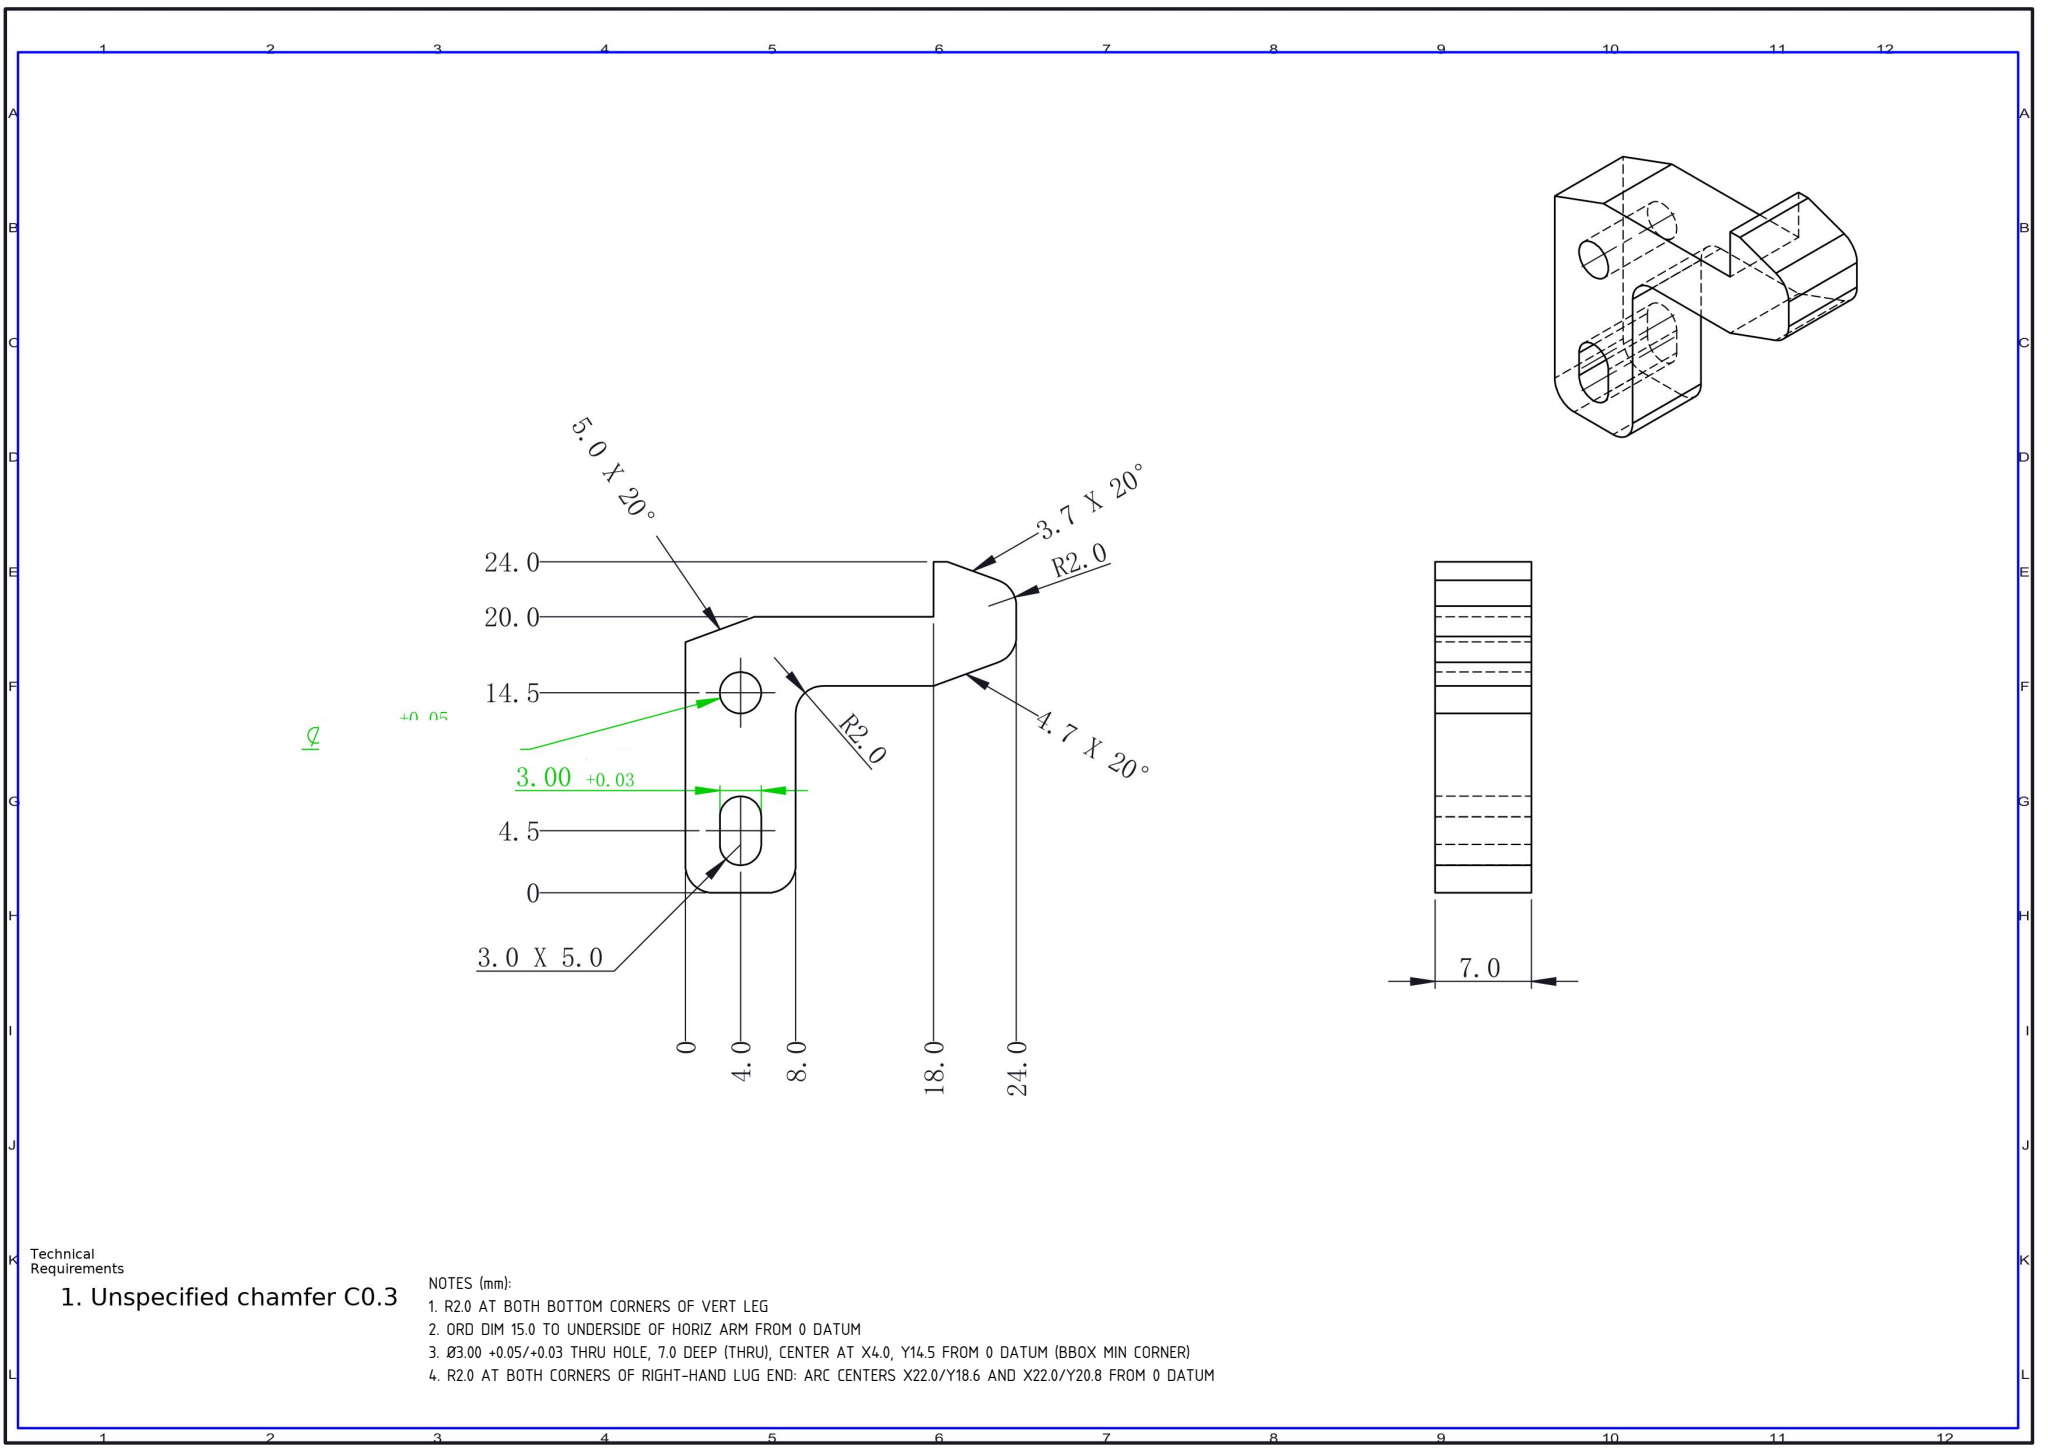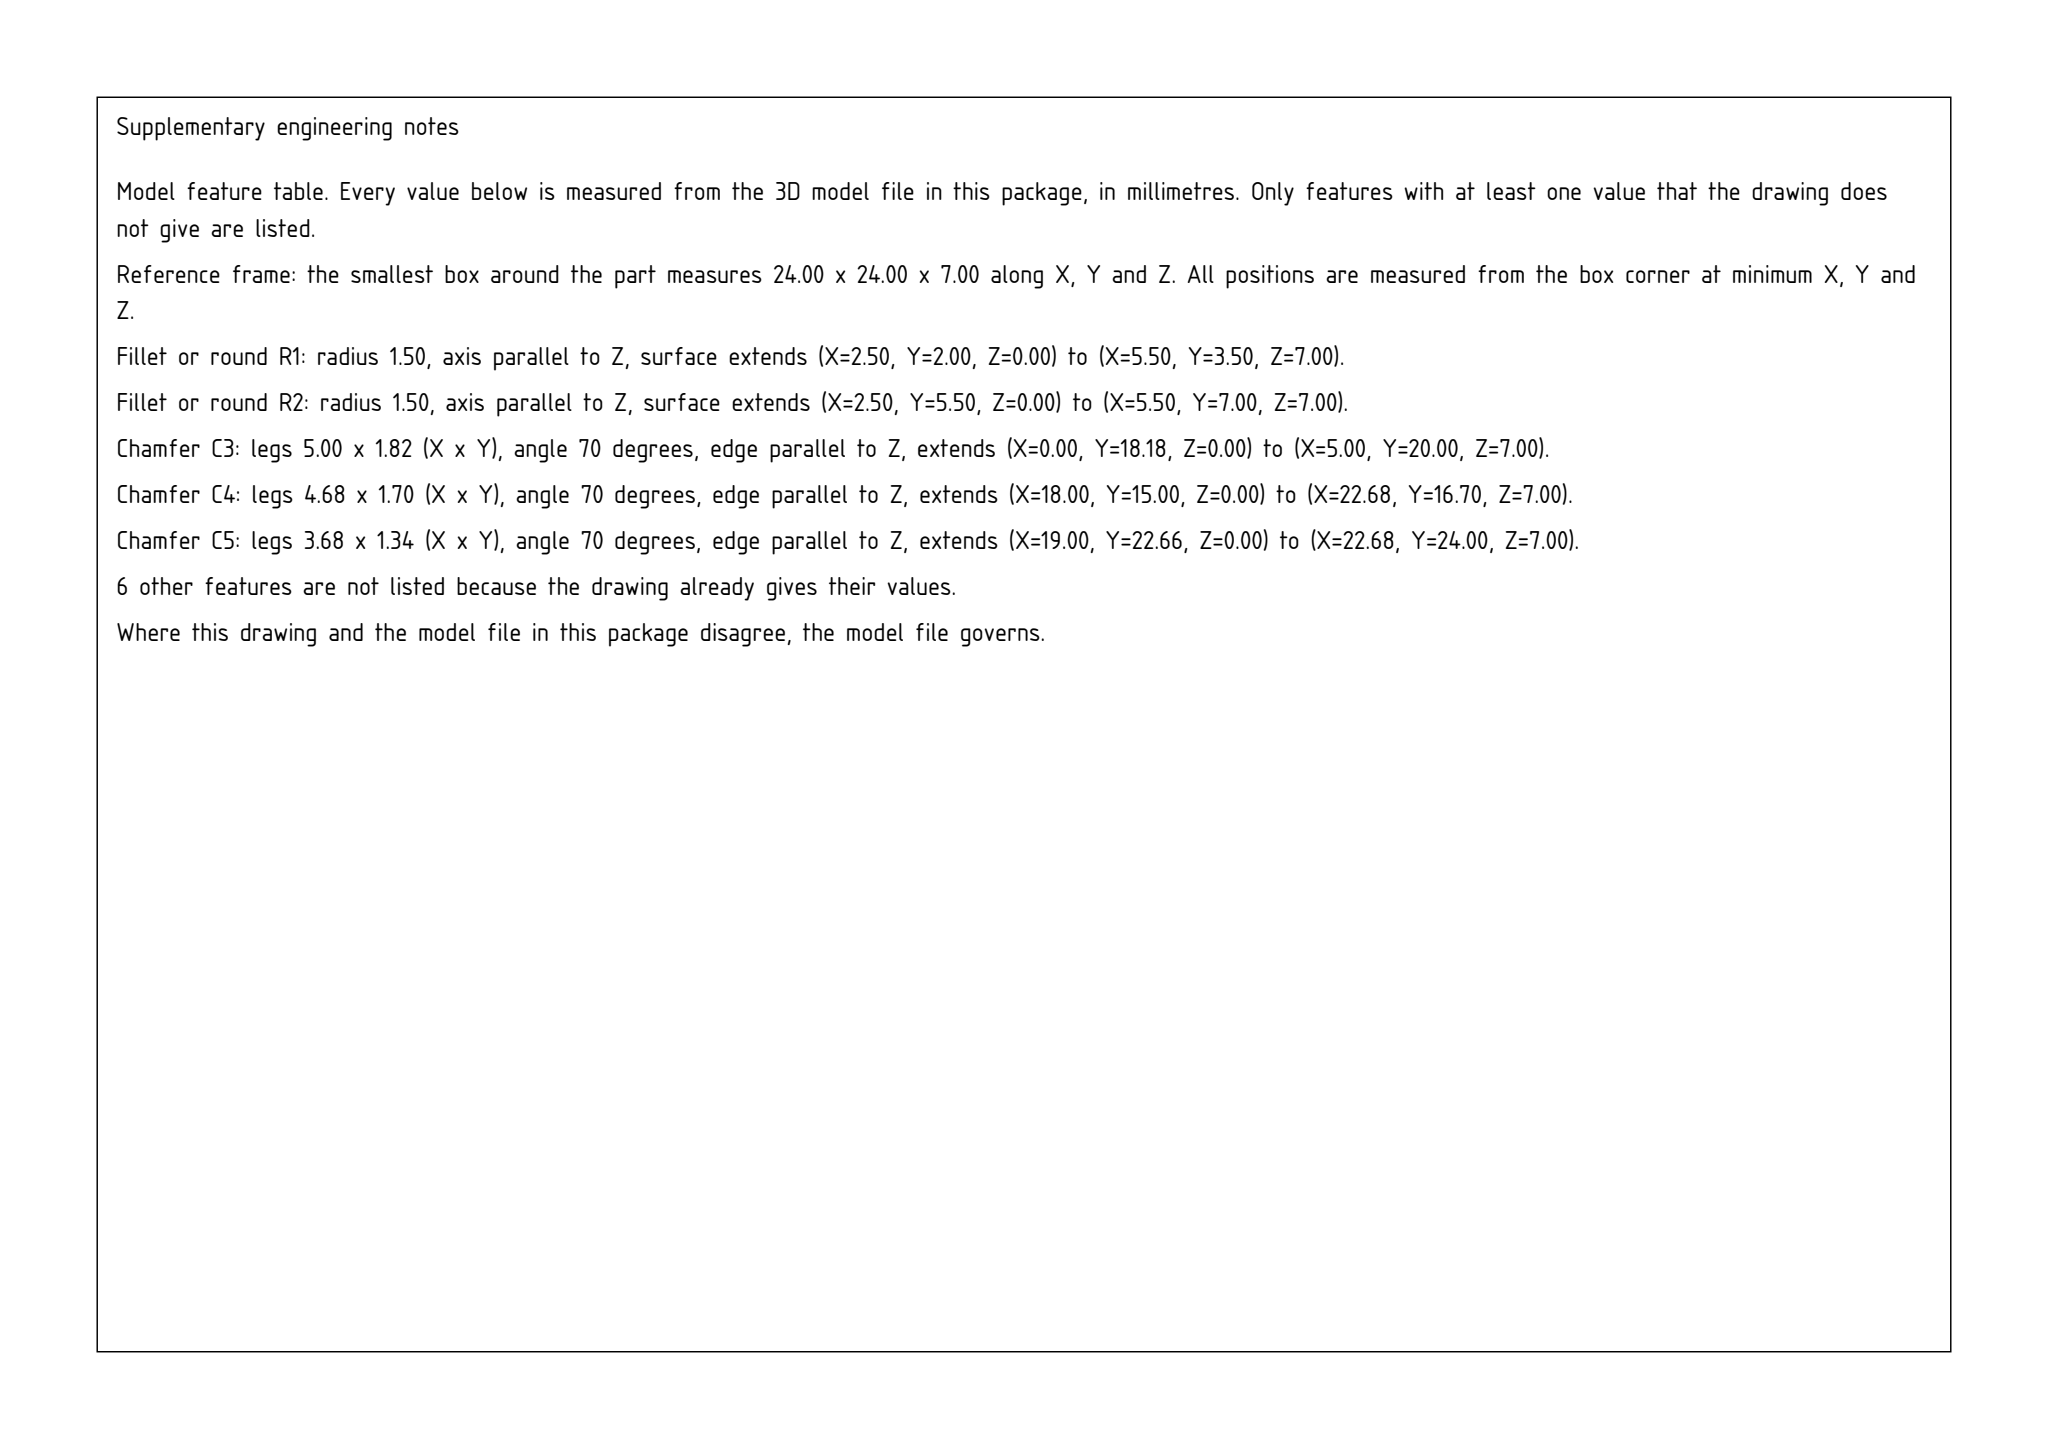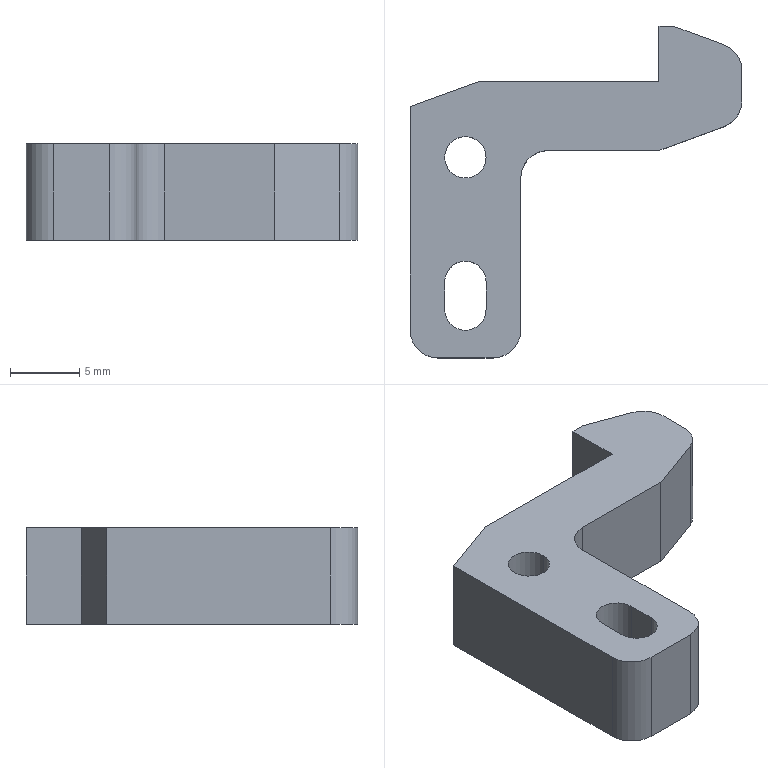Part | SolidWorks | mm | 1 solid | 24 faces | box 24 x 24 x 7 mm | volume 1586 mm3 | plane 15 | cylinder 9 | commonest cylinder face diameters 4 x5 3 x4
Drawing notes:
R2.0 AT BOTH BOTTOM CORNERS OF VERT LEG | from the solid: 4.0 dia z-cylinders at (2.0,2.0) and (6.0,2.0) => R2.0 corner fillets
ORD DIM 15.0 TO UNDERSIDE OF HORIZ ARM FROM 0 DATUM | from the solid: y-normal plane at offset 15.0 (bottom face of arm), datum y=0
Ø3.00 +0.05/+0.03 THRU HOLE, 7.0 DEEP (THRU), CENTER AT X4.0, Y14.5 FROM 0 DATUM (BBOX MIN CORNER) | from the solid: cylinders: hole/bore, dia 3.0, axis z at [4.0, 14.5], from 0.0 to 7.0, 360 deg
R2.0 AT BOTH CORNERS OF RIGHT-HAND LUG END: ARC CENTERS X22.0/Y18.6 AND X22.0/Y20.8 FROM 0 DATUM | from the solid: cylinders: convex arc dia 4.0, axis z at [22.0, 18.6] and [22.0, 20.8], each 70 deg, from 0.0 to 7.0
build123d program:
from build123d import *

# Parameters (mm, degrees)
BOSS_EXTRUDE1_DEPTH = 7
FILLET1_R           = 2
SKETCH2_R           = 1.5
CUT_EXTRUDE1_DEPTH  = 35.655
CHAMFER1_SIZE       = 5
CHAMFER1_SIZE2      = 1.82
CUT_EXTRUDE2_DEPTH  = 35.655
FILLET3_R           = 2


with BuildPart() as part:
    # Sketch1 → Boss-Extrude1 (new body)
    with BuildSketch(Plane.XY):
        Polygon((19, 24), (24, 22.18), (24, 17.184), (18, 15), (8, 15), (8, 0), (0, 0), (0, 20), (18, 20), (18, 24), align=None)
    extrude(amount=BOSS_EXTRUDE1_DEPTH)

    # Fillet1
    fillet1_edges = [part.edges().sort_by_distance(p)[0] for p in [
        (8, 15, 3.5),
    ]]
    fillet(fillet1_edges, radius=FILLET1_R)

    # Sketch2 → Cut-Extrude1 (cut, through all)
    with BuildSketch(Plane(origin=(0, 0, 0), x_dir=(-1, 0, 0), z_dir=(0, 0, -1))):
        with Locations((-4, 14.5)):
            Circle(SKETCH2_R)
    extrude(amount=-CUT_EXTRUDE1_DEPTH, mode=Mode.SUBTRACT)

    # Chamfer1
    chamfer1_edges = [part.edges().sort_by_distance(p)[0] for p in [
        (0, 20, 3.5),
    ]]
    chamfer1_side = [part.faces().sort_by_distance(p)[0] for p in [
        (9, 20, 3.5),
    ]]
    chamfer(chamfer1_edges, length=CHAMFER1_SIZE, length2=CHAMFER1_SIZE2, reference=chamfer1_side[0])

    # Sketch3 → Cut-Extrude2 (cut, through all)
    with BuildSketch(Plane(origin=(0, 0, 0), x_dir=(-1, 0, 0), z_dir=(0, 0, -1))):
        with BuildLine():
            Line((-2.5, 5.5), (-2.5, 3.5))
            ThreePointArc((-2.5, 3.5), (-4, 2), (-5.5, 3.5))
            Line((-5.5, 3.5), (-5.5, 5.5))
            ThreePointArc((-5.5, 5.5), (-4, 7), (-2.5, 5.5))
        make_face()
    extrude(amount=-CUT_EXTRUDE2_DEPTH, mode=Mode.SUBTRACT)

    # Fillet3
    fillet3_edges = [part.edges().sort_by_distance(p)[0] for p in [
        (24, 22.18, 3.5),
        (24, 17.184, 3.5),
        (8, 0, 3.5),
        (0, 0, 3.5),
    ]]
    fillet(fillet3_edges, radius=FILLET3_R)


solid = part.part
STEP:
#1=CARTESIAN_POINT('',(5.5,14.5,7.));
#2=VERTEX_POINT('',#1);
#3=CARTESIAN_POINT('',(2.5,14.5,7.));
#4=VERTEX_POINT('',#3);
#5=CARTESIAN_POINT('',(4.,14.5,7.));
#6=DIRECTION('',(0.,0.,-1.));
#7=DIRECTION('',(-1.,0.,0.));
#8=AXIS2_PLACEMENT_3D('',#5,#6,#7);
#9=CIRCLE('',#8,1.5);
#10=EDGE_CURVE('',#2,#4,#9,.T.);
#11=ORIENTED_EDGE('',*,*,#10,.F.);
#12=CARTESIAN_POINT('',(5.5,14.5,0.));
#13=VERTEX_POINT('',#12);
#14=CARTESIAN_POINT('',(5.5,14.5,7.));
#15=DIRECTION('',(0.,0.,-1.));
#16=VECTOR('',#15,1000.);
#17=LINE('',#14,#16);
#18=EDGE_CURVE('',#2,#13,#17,.T.);
#19=ORIENTED_EDGE('',*,*,#18,.T.);
#20=CARTESIAN_POINT('',(2.5,14.5,0.));
#21=VERTEX_POINT('',#20);
#22=CARTESIAN_POINT('',(4.,14.5,0.));
#23=DIRECTION('',(0.,0.,-1.));
#24=DIRECTION('',(-1.,0.,0.));
#25=AXIS2_PLACEMENT_3D('',#22,#23,#24);
#26=CIRCLE('',#25,1.5);
#27=EDGE_CURVE('',#13,#21,#26,.T.);
#28=ORIENTED_EDGE('',*,*,#27,.T.);
#29=CARTESIAN_POINT('',(2.5,14.5,7.));
#30=DIRECTION('',(0.,0.,-1.));
#31=VECTOR('',#30,1000.);
#32=LINE('',#29,#31);
#33=EDGE_CURVE('',#4,#21,#32,.T.);
#34=ORIENTED_EDGE('',*,*,#33,.F.);
#35=EDGE_LOOP('',(#11,#19,#28,#34));
#36=FACE_OUTER_BOUND('',#35,.T.);
#37=CARTESIAN_POINT('',(4.,14.5,7.));
#38=DIRECTION('',(0.,0.,-1.));
#39=DIRECTION('',(-1.,0.,0.));
#40=AXIS2_PLACEMENT_3D('',#37,#38,#39);
#41=CYLINDRICAL_SURFACE('',#40,1.5);
#42=ADVANCED_FACE('',(#36),#41,.F.);
#43=CARTESIAN_POINT('',(0.,18.18,0.));
#44=VERTEX_POINT('',#43);
#45=CARTESIAN_POINT('',(0.,2.,0.));
#46=VERTEX_POINT('',#45);
#47=CARTESIAN_POINT('',(0.,0.,0.));
#48=DIRECTION('',(0.,-1.,0.));
#49=VECTOR('',#48,1000.);
#50=LINE('',#47,#49);
#51=EDGE_CURVE('',#44,#46,#50,.T.);
#52=ORIENTED_EDGE('',*,*,#51,.T.);
#53=CARTESIAN_POINT('',(0.,2.,7.));
#54=VERTEX_POINT('',#53);
#55=CARTESIAN_POINT('',(0.,2.,7.));
#56=DIRECTION('',(0.,0.,1.));
#57=VECTOR('',#56,1000.);
#58=LINE('',#55,#57);
#59=EDGE_CURVE('',#46,#54,#58,.T.);
#60=ORIENTED_EDGE('',*,*,#59,.T.);
#61=CARTESIAN_POINT('',(0.,18.18,7.));
#62=VERTEX_POINT('',#61);
#63=CARTESIAN_POINT('',(0.,0.,7.));
#64=DIRECTION('',(0.,-1.,0.));
#65=VECTOR('',#64,1000.);
#66=LINE('',#63,#65);
#67=EDGE_CURVE('',#62,#54,#66,.T.);
#68=ORIENTED_EDGE('',*,*,#67,.F.);
#69=CARTESIAN_POINT('',(0.,18.18,7.));
#70=DIRECTION('',(0.,0.,-1.));
#71=VECTOR('',#70,1000.);
#72=LINE('',#69,#71);
#73=EDGE_CURVE('',#62,#44,#72,.T.);
#74=ORIENTED_EDGE('',*,*,#73,.T.);
#75=EDGE_LOOP('',(#52,#60,#68,#74));
#76=FACE_OUTER_BOUND('',#75,.T.);
#77=CARTESIAN_POINT('',(0.,0.,7.));
#78=DIRECTION('',(1.,0.,0.));
#79=DIRECTION('',(0.,0.,-1.));
#80=AXIS2_PLACEMENT_3D('',#77,#78,#79);
#81=PLANE('',#80);
#82=ADVANCED_FACE('',(#76),#81,.F.);
#83=CARTESIAN_POINT('',(2.,0.,7.));
#84=VERTEX_POINT('',#83);
#85=CARTESIAN_POINT('',(6.,0.,7.));
#86=VERTEX_POINT('',#85);
#87=CARTESIAN_POINT('',(0.,0.,7.));
#88=DIRECTION('',(1.,0.,0.));
#89=VECTOR('',#88,1000.);
#90=LINE('',#87,#89);
#91=EDGE_CURVE('',#84,#86,#90,.T.);
#92=ORIENTED_EDGE('',*,*,#91,.F.);
#93=CARTESIAN_POINT('',(2.,0.,0.));
#94=VERTEX_POINT('',#93);
#95=CARTESIAN_POINT('',(2.,0.,7.));
#96=DIRECTION('',(0.,0.,-1.));
#97=VECTOR('',#96,1000.);
#98=LINE('',#95,#97);
#99=EDGE_CURVE('',#84,#94,#98,.T.);
#100=ORIENTED_EDGE('',*,*,#99,.T.);
#101=CARTESIAN_POINT('',(6.,0.,0.));
#102=VERTEX_POINT('',#101);
#103=CARTESIAN_POINT('',(0.,0.,0.));
#104=DIRECTION('',(1.,0.,0.));
#105=VECTOR('',#104,1000.);
#106=LINE('',#103,#105);
#107=EDGE_CURVE('',#94,#102,#106,.T.);
#108=ORIENTED_EDGE('',*,*,#107,.T.);
#109=CARTESIAN_POINT('',(6.,0.,7.));
#110=DIRECTION('',(0.,0.,1.));
#111=VECTOR('',#110,1000.);
#112=LINE('',#109,#111);
#113=EDGE_CURVE('',#102,#86,#112,.T.);
#114=ORIENTED_EDGE('',*,*,#113,.T.);
#115=EDGE_LOOP('',(#92,#100,#108,#114));
#116=FACE_OUTER_BOUND('',#115,.T.);
#117=CARTESIAN_POINT('',(0.,0.,7.));
#118=DIRECTION('',(0.,1.,0.));
#119=DIRECTION('',(0.,0.,1.));
#120=AXIS2_PLACEMENT_3D('',#117,#118,#119);
#121=PLANE('',#120);
#122=ADVANCED_FACE('',(#116),#121,.F.);
#123=CARTESIAN_POINT('',(8.,2.,7.));
#124=VERTEX_POINT('',#123);
#125=CARTESIAN_POINT('',(8.,13.,7.));
#126=VERTEX_POINT('',#125);
#127=CARTESIAN_POINT('',(8.,0.,7.));
#128=DIRECTION('',(0.,1.,0.));
#129=VECTOR('',#128,1000.);
#130=LINE('',#127,#129);
#131=EDGE_CURVE('',#124,#126,#130,.T.);
#132=ORIENTED_EDGE('',*,*,#131,.F.);
#133=CARTESIAN_POINT('',(8.,2.,0.));
#134=VERTEX_POINT('',#133);
#135=CARTESIAN_POINT('',(8.,2.,7.));
#136=DIRECTION('',(0.,0.,-1.));
#137=VECTOR('',#136,1000.);
#138=LINE('',#135,#137);
#139=EDGE_CURVE('',#124,#134,#138,.T.);
#140=ORIENTED_EDGE('',*,*,#139,.T.);
#141=CARTESIAN_POINT('',(8.,13.,0.));
#142=VERTEX_POINT('',#141);
#143=CARTESIAN_POINT('',(8.,0.,0.));
#144=DIRECTION('',(0.,1.,0.));
#145=VECTOR('',#144,1000.);
#146=LINE('',#143,#145);
#147=EDGE_CURVE('',#134,#142,#146,.T.);
#148=ORIENTED_EDGE('',*,*,#147,.T.);
#149=CARTESIAN_POINT('',(8.,13.,7.));
#150=DIRECTION('',(0.,0.,1.));
#151=VECTOR('',#150,1000.);
#152=LINE('',#149,#151);
#153=EDGE_CURVE('',#142,#126,#152,.T.);
#154=ORIENTED_EDGE('',*,*,#153,.T.);
#155=EDGE_LOOP('',(#132,#140,#148,#154));
#156=FACE_OUTER_BOUND('',#155,.T.);
#157=CARTESIAN_POINT('',(8.,0.,7.));
#158=DIRECTION('',(-1.,0.,0.));
#159=DIRECTION('',(0.,0.,1.));
#160=AXIS2_PLACEMENT_3D('',#157,#158,#159);
#161=PLANE('',#160);
#162=ADVANCED_FACE('',(#156),#161,.F.);
#163=CARTESIAN_POINT('',(10.,15.,7.));
#164=VERTEX_POINT('',#163);
#165=CARTESIAN_POINT('',(18.,15.,7.));
#166=VERTEX_POINT('',#165);
#167=CARTESIAN_POINT('',(18.,15.,7.));
#168=DIRECTION('',(1.,0.,0.));
#169=VECTOR('',#168,1000.);
#170=LINE('',#167,#169);
#171=EDGE_CURVE('',#164,#166,#170,.T.);
#172=ORIENTED_EDGE('',*,*,#171,.F.);
#173=CARTESIAN_POINT('',(10.,15.,0.));
#174=VERTEX_POINT('',#173);
#175=CARTESIAN_POINT('',(10.,15.,0.));
#176=DIRECTION('',(0.,0.,-1.));
#177=VECTOR('',#176,1000.);
#178=LINE('',#175,#177);
#179=EDGE_CURVE('',#164,#174,#178,.T.);
#180=ORIENTED_EDGE('',*,*,#179,.T.);
#181=CARTESIAN_POINT('',(18.,15.,0.));
#182=VERTEX_POINT('',#181);
#183=CARTESIAN_POINT('',(18.,15.,0.));
#184=DIRECTION('',(1.,0.,0.));
#185=VECTOR('',#184,1000.);
#186=LINE('',#183,#185);
#187=EDGE_CURVE('',#174,#182,#186,.T.);
#188=ORIENTED_EDGE('',*,*,#187,.T.);
#189=CARTESIAN_POINT('',(18.,15.,7.));
#190=DIRECTION('',(0.,0.,-1.));
#191=VECTOR('',#190,1000.);
#192=LINE('',#189,#191);
#193=EDGE_CURVE('',#166,#182,#192,.T.);
#194=ORIENTED_EDGE('',*,*,#193,.F.);
#195=EDGE_LOOP('',(#172,#180,#188,#194));
#196=FACE_OUTER_BOUND('',#195,.T.);
#197=CARTESIAN_POINT('',(18.,15.,7.));
#198=DIRECTION('',(-0.,1.,0.));
#199=DIRECTION('',(-1.,-0.,0.));
#200=AXIS2_PLACEMENT_3D('',#197,#198,#199);
#201=PLANE('',#200);
#202=ADVANCED_FACE('',(#196),#201,.F.);
#203=CARTESIAN_POINT('',(22.684,16.705,0.));
#204=VERTEX_POINT('',#203);
#205=CARTESIAN_POINT('',(24.,17.184,0.));
#206=DIRECTION('',(0.9397,0.342,0.));
#207=VECTOR('',#206,1000.);
#208=LINE('',#205,#207);
#209=EDGE_CURVE('',#182,#204,#208,.T.);
#210=ORIENTED_EDGE('',*,*,#209,.T.);
#211=CARTESIAN_POINT('',(22.684,16.705,7.));
#212=VERTEX_POINT('',#211);
#213=CARTESIAN_POINT('',(22.684,16.705,7.));
#214=DIRECTION('',(0.,0.,1.));
#215=VECTOR('',#214,1000.);
#216=LINE('',#213,#215);
#217=EDGE_CURVE('',#204,#212,#216,.T.);
#218=ORIENTED_EDGE('',*,*,#217,.T.);
#219=CARTESIAN_POINT('',(24.,17.184,7.));
#220=DIRECTION('',(0.9397,0.342,0.));
#221=VECTOR('',#220,1000.);
#222=LINE('',#219,#221);
#223=EDGE_CURVE('',#166,#212,#222,.T.);
#224=ORIENTED_EDGE('',*,*,#223,.F.);
#225=ORIENTED_EDGE('',*,*,#193,.T.);
#226=EDGE_LOOP('',(#210,#218,#224,#225));
#227=FACE_OUTER_BOUND('',#226,.T.);
#228=CARTESIAN_POINT('',(24.,17.184,7.));
#229=DIRECTION('',(-0.342,0.9397,0.));
#230=DIRECTION('',(-0.9397,-0.342,0.));
#231=AXIS2_PLACEMENT_3D('',#228,#229,#230);
#232=PLANE('',#231);
#233=ADVANCED_FACE('',(#227),#232,.F.);
#234=CARTESIAN_POINT('',(24.,18.584,7.));
#235=VERTEX_POINT('',#234);
#236=CARTESIAN_POINT('',(24.,20.78,7.));
#237=VERTEX_POINT('',#236);
#238=CARTESIAN_POINT('',(24.,17.184,7.));
#239=DIRECTION('',(0.,1.,0.));
#240=VECTOR('',#239,1000.);
#241=LINE('',#238,#240);
#242=EDGE_CURVE('',#235,#237,#241,.T.);
#243=ORIENTED_EDGE('',*,*,#242,.F.);
#244=CARTESIAN_POINT('',(24.,18.584,0.));
#245=VERTEX_POINT('',#244);
#246=CARTESIAN_POINT('',(24.,18.584,7.));
#247=DIRECTION('',(0.,0.,-1.));
#248=VECTOR('',#247,1000.);
#249=LINE('',#246,#248);
#250=EDGE_CURVE('',#235,#245,#249,.T.);
#251=ORIENTED_EDGE('',*,*,#250,.T.);
#252=CARTESIAN_POINT('',(24.,20.78,0.));
#253=VERTEX_POINT('',#252);
#254=CARTESIAN_POINT('',(24.,17.184,0.));
#255=DIRECTION('',(0.,1.,0.));
#256=VECTOR('',#255,1000.);
#257=LINE('',#254,#256);
#258=EDGE_CURVE('',#245,#253,#257,.T.);
#259=ORIENTED_EDGE('',*,*,#258,.T.);
#260=CARTESIAN_POINT('',(24.,20.78,7.));
#261=DIRECTION('',(0.,0.,1.));
#262=VECTOR('',#261,1000.);
#263=LINE('',#260,#262);
#264=EDGE_CURVE('',#253,#237,#263,.T.);
#265=ORIENTED_EDGE('',*,*,#264,.T.);
#266=EDGE_LOOP('',(#243,#251,#259,#265));
#267=FACE_OUTER_BOUND('',#266,.T.);
#268=CARTESIAN_POINT('',(24.,17.184,7.));
#269=DIRECTION('',(-1.,0.,0.));
#270=DIRECTION('',(0.,0.,1.));
#271=AXIS2_PLACEMENT_3D('',#268,#269,#270);
#272=PLANE('',#271);
#273=ADVANCED_FACE('',(#267),#272,.F.);
#274=CARTESIAN_POINT('',(22.684,22.659,7.));
#275=VERTEX_POINT('',#274);
#276=CARTESIAN_POINT('',(19.,24.,7.));
#277=VERTEX_POINT('',#276);
#278=CARTESIAN_POINT('',(19.,24.,7.));
#279=DIRECTION('',(-0.9397,0.342,0.));
#280=VECTOR('',#279,1000.);
#281=LINE('',#278,#280);
#282=EDGE_CURVE('',#275,#277,#281,.T.);
#283=ORIENTED_EDGE('',*,*,#282,.F.);
#284=CARTESIAN_POINT('',(22.684,22.659,0.));
#285=VERTEX_POINT('',#284);
#286=CARTESIAN_POINT('',(22.684,22.659,7.));
#287=DIRECTION('',(0.,0.,-1.));
#288=VECTOR('',#287,1000.);
#289=LINE('',#286,#288);
#290=EDGE_CURVE('',#275,#285,#289,.T.);
#291=ORIENTED_EDGE('',*,*,#290,.T.);
#292=CARTESIAN_POINT('',(19.,24.,0.));
#293=VERTEX_POINT('',#292);
#294=CARTESIAN_POINT('',(19.,24.,0.));
#295=DIRECTION('',(-0.9397,0.342,0.));
#296=VECTOR('',#295,1000.);
#297=LINE('',#294,#296);
#298=EDGE_CURVE('',#285,#293,#297,.T.);
#299=ORIENTED_EDGE('',*,*,#298,.T.);
#300=CARTESIAN_POINT('',(19.,24.,7.));
#301=DIRECTION('',(0.,0.,-1.));
#302=VECTOR('',#301,1000.);
#303=LINE('',#300,#302);
#304=EDGE_CURVE('',#277,#293,#303,.T.);
#305=ORIENTED_EDGE('',*,*,#304,.F.);
#306=EDGE_LOOP('',(#283,#291,#299,#305));
#307=FACE_OUTER_BOUND('',#306,.T.);
#308=CARTESIAN_POINT('',(19.,24.,7.));
#309=DIRECTION('',(-0.342,-0.9397,0.));
#310=DIRECTION('',(0.9397,-0.342,0.));
#311=AXIS2_PLACEMENT_3D('',#308,#309,#310);
#312=PLANE('',#311);
#313=ADVANCED_FACE('',(#307),#312,.F.);
#314=CARTESIAN_POINT('',(18.,24.,0.));
#315=VERTEX_POINT('',#314);
#316=CARTESIAN_POINT('',(18.,24.,0.));
#317=DIRECTION('',(-1.,0.,0.));
#318=VECTOR('',#317,1000.);
#319=LINE('',#316,#318);
#320=EDGE_CURVE('',#293,#315,#319,.T.);
#321=ORIENTED_EDGE('',*,*,#320,.T.);
#322=CARTESIAN_POINT('',(18.,24.,7.));
#323=VERTEX_POINT('',#322);
#324=CARTESIAN_POINT('',(18.,24.,7.));
#325=DIRECTION('',(0.,0.,-1.));
#326=VECTOR('',#325,1000.);
#327=LINE('',#324,#326);
#328=EDGE_CURVE('',#323,#315,#327,.T.);
#329=ORIENTED_EDGE('',*,*,#328,.F.);
#330=CARTESIAN_POINT('',(18.,24.,7.));
#331=DIRECTION('',(-1.,0.,0.));
#332=VECTOR('',#331,1000.);
#333=LINE('',#330,#332);
#334=EDGE_CURVE('',#277,#323,#333,.T.);
#335=ORIENTED_EDGE('',*,*,#334,.F.);
#336=ORIENTED_EDGE('',*,*,#304,.T.);
#337=EDGE_LOOP('',(#321,#329,#335,#336));
#338=FACE_OUTER_BOUND('',#337,.T.);
#339=CARTESIAN_POINT('',(18.,24.,7.));
#340=DIRECTION('',(0.,-1.,0.));
#341=DIRECTION('',(0.,0.,-1.));
#342=AXIS2_PLACEMENT_3D('',#339,#340,#341);
#343=PLANE('',#342);
#344=ADVANCED_FACE('',(#338),#343,.F.);
#345=CARTESIAN_POINT('',(18.,20.,0.));
#346=VERTEX_POINT('',#345);
#347=CARTESIAN_POINT('',(18.,24.,0.));
#348=DIRECTION('',(0.,-1.,0.));
#349=VECTOR('',#348,1000.);
#350=LINE('',#347,#349);
#351=EDGE_CURVE('',#315,#346,#350,.T.);
#352=ORIENTED_EDGE('',*,*,#351,.T.);
#353=CARTESIAN_POINT('',(18.,20.,7.));
#354=VERTEX_POINT('',#353);
#355=CARTESIAN_POINT('',(18.,20.,7.));
#356=DIRECTION('',(0.,0.,-1.));
#357=VECTOR('',#356,1000.);
#358=LINE('',#355,#357);
#359=EDGE_CURVE('',#354,#346,#358,.T.);
#360=ORIENTED_EDGE('',*,*,#359,.F.);
#361=CARTESIAN_POINT('',(18.,24.,7.));
#362=DIRECTION('',(0.,-1.,0.));
#363=VECTOR('',#362,1000.);
#364=LINE('',#361,#363);
#365=EDGE_CURVE('',#323,#354,#364,.T.);
#366=ORIENTED_EDGE('',*,*,#365,.F.);
#367=ORIENTED_EDGE('',*,*,#328,.T.);
#368=EDGE_LOOP('',(#352,#360,#366,#367));
#369=FACE_OUTER_BOUND('',#368,.T.);
#370=CARTESIAN_POINT('',(18.,24.,7.));
#371=DIRECTION('',(1.,0.,0.));
#372=DIRECTION('',(0.,0.,-1.));
#373=AXIS2_PLACEMENT_3D('',#370,#371,#372);
#374=PLANE('',#373);
#375=ADVANCED_FACE('',(#369),#374,.F.);
#376=CARTESIAN_POINT('',(5.,20.,0.));
#377=VERTEX_POINT('',#376);
#378=CARTESIAN_POINT('',(0.,20.,0.));
#379=DIRECTION('',(-1.,0.,0.));
#380=VECTOR('',#379,1000.);
#381=LINE('',#378,#380);
#382=EDGE_CURVE('',#346,#377,#381,.T.);
#383=ORIENTED_EDGE('',*,*,#382,.T.);
#384=CARTESIAN_POINT('',(5.,20.,7.));
#385=VERTEX_POINT('',#384);
#386=CARTESIAN_POINT('',(5.,20.,7.));
#387=DIRECTION('',(0.,0.,1.));
#388=VECTOR('',#387,1000.);
#389=LINE('',#386,#388);
#390=EDGE_CURVE('',#377,#385,#389,.T.);
#391=ORIENTED_EDGE('',*,*,#390,.T.);
#392=CARTESIAN_POINT('',(0.,20.,7.));
#393=DIRECTION('',(-1.,0.,0.));
#394=VECTOR('',#393,1000.);
#395=LINE('',#392,#394);
#396=EDGE_CURVE('',#354,#385,#395,.T.);
#397=ORIENTED_EDGE('',*,*,#396,.F.);
#398=ORIENTED_EDGE('',*,*,#359,.T.);
#399=EDGE_LOOP('',(#383,#391,#397,#398));
#400=FACE_OUTER_BOUND('',#399,.T.);
#401=CARTESIAN_POINT('',(0.,20.,7.));
#402=DIRECTION('',(0.,-1.,0.));
#403=DIRECTION('',(0.,0.,-1.));
#404=AXIS2_PLACEMENT_3D('',#401,#402,#403);
#405=PLANE('',#404);
#406=ADVANCED_FACE('',(#400),#405,.F.);
#407=CARTESIAN_POINT('',(2.5,3.5,7.));
#408=VERTEX_POINT('',#407);
#409=CARTESIAN_POINT('',(2.5,5.5,7.));
#410=VERTEX_POINT('',#409);
#411=CARTESIAN_POINT('',(2.5,5.5,7.));
#412=DIRECTION('',(0.,1.,0.));
#413=VECTOR('',#412,1000.);
#414=LINE('',#411,#413);
#415=EDGE_CURVE('',#408,#410,#414,.T.);
#416=ORIENTED_EDGE('',*,*,#415,.T.);
#417=CARTESIAN_POINT('',(5.5,5.5,7.));
#418=VERTEX_POINT('',#417);
#419=CARTESIAN_POINT('',(4.,5.5,7.));
#420=DIRECTION('',(0.,0.,-1.));
#421=DIRECTION('',(-1.,0.,0.));
#422=AXIS2_PLACEMENT_3D('',#419,#420,#421);
#423=CIRCLE('',#422,1.5);
#424=EDGE_CURVE('',#410,#418,#423,.T.);
#425=ORIENTED_EDGE('',*,*,#424,.T.);
#426=CARTESIAN_POINT('',(5.5,3.5,7.));
#427=VERTEX_POINT('',#426);
#428=CARTESIAN_POINT('',(5.5,5.5,7.));
#429=DIRECTION('',(-0.,-1.,0.));
#430=VECTOR('',#429,1000.);
#431=LINE('',#428,#430);
#432=EDGE_CURVE('',#418,#427,#431,.T.);
#433=ORIENTED_EDGE('',*,*,#432,.T.);
#434=CARTESIAN_POINT('',(4.,3.5,7.));
#435=DIRECTION('',(0.,0.,-1.));
#436=DIRECTION('',(-1.,0.,0.));
#437=AXIS2_PLACEMENT_3D('',#434,#435,#436);
#438=CIRCLE('',#437,1.5);
#439=EDGE_CURVE('',#427,#408,#438,.T.);
#440=ORIENTED_EDGE('',*,*,#439,.T.);
#441=EDGE_LOOP('',(#416,#425,#433,#440));
#442=FACE_BOUND('',#441,.T.);
#443=CARTESIAN_POINT('',(4.,14.5,7.));
#444=DIRECTION('',(0.,0.,-1.));
#445=DIRECTION('',(-1.,0.,0.));
#446=AXIS2_PLACEMENT_3D('',#443,#444,#445);
#447=CIRCLE('',#446,1.5);
#448=EDGE_CURVE('',#4,#2,#447,.T.);
#449=ORIENTED_EDGE('',*,*,#448,.T.);
#450=ORIENTED_EDGE('',*,*,#10,.T.);
#451=EDGE_LOOP('',(#449,#450));
#452=FACE_BOUND('',#451,.T.);
#453=ORIENTED_EDGE('',*,*,#67,.T.);
#454=CARTESIAN_POINT('',(2.,2.,7.));
#455=DIRECTION('',(0.,0.,1.));
#456=DIRECTION('',(-1.,0.,0.));
#457=AXIS2_PLACEMENT_3D('',#454,#455,#456);
#458=CIRCLE('',#457,2.);
#459=EDGE_CURVE('',#54,#84,#458,.T.);
#460=ORIENTED_EDGE('',*,*,#459,.T.);
#461=ORIENTED_EDGE('',*,*,#91,.T.);
#462=CARTESIAN_POINT('',(6.,2.,7.));
#463=DIRECTION('',(0.,0.,1.));
#464=DIRECTION('',(-1.,0.,0.));
#465=AXIS2_PLACEMENT_3D('',#462,#463,#464);
#466=CIRCLE('',#465,2.);
#467=EDGE_CURVE('',#86,#124,#466,.T.);
#468=ORIENTED_EDGE('',*,*,#467,.T.);
#469=ORIENTED_EDGE('',*,*,#131,.T.);
#470=CARTESIAN_POINT('',(10.,13.,7.));
#471=DIRECTION('',(0.,0.,-1.));
#472=DIRECTION('',(-1.,0.,0.));
#473=AXIS2_PLACEMENT_3D('',#470,#471,#472);
#474=CIRCLE('',#473,2.);
#475=EDGE_CURVE('',#126,#164,#474,.T.);
#476=ORIENTED_EDGE('',*,*,#475,.T.);
#477=ORIENTED_EDGE('',*,*,#171,.T.);
#478=ORIENTED_EDGE('',*,*,#223,.T.);
#479=CARTESIAN_POINT('',(22.,18.584,7.));
#480=DIRECTION('',(0.,0.,1.));
#481=DIRECTION('',(-1.,0.,0.));
#482=AXIS2_PLACEMENT_3D('',#479,#480,#481);
#483=CIRCLE('',#482,2.);
#484=EDGE_CURVE('',#212,#235,#483,.T.);
#485=ORIENTED_EDGE('',*,*,#484,.T.);
#486=ORIENTED_EDGE('',*,*,#242,.T.);
#487=CARTESIAN_POINT('',(22.,20.78,7.));
#488=DIRECTION('',(0.,0.,1.));
#489=DIRECTION('',(-1.,0.,0.));
#490=AXIS2_PLACEMENT_3D('',#487,#488,#489);
#491=CIRCLE('',#490,2.);
#492=EDGE_CURVE('',#237,#275,#491,.T.);
#493=ORIENTED_EDGE('',*,*,#492,.T.);
#494=ORIENTED_EDGE('',*,*,#282,.T.);
#495=ORIENTED_EDGE('',*,*,#334,.T.);
#496=ORIENTED_EDGE('',*,*,#365,.T.);
#497=ORIENTED_EDGE('',*,*,#396,.T.);
#498=CARTESIAN_POINT('',(0.,18.18,7.));
#499=DIRECTION('',(-0.9397,-0.342,0.));
#500=VECTOR('',#499,1000.);
#501=LINE('',#498,#500);
#502=EDGE_CURVE('',#385,#62,#501,.T.);
#503=ORIENTED_EDGE('',*,*,#502,.T.);
#504=EDGE_LOOP('',(#453,#460,#461,#468,#469,#476,#477,#478,#485,#486,#493,#494,#495,#496,#497,#503));
#505=FACE_OUTER_BOUND('',#504,.T.);
#506=CARTESIAN_POINT('',(0.,0.,7.));
#507=DIRECTION('',(0.,0.,-1.));
#508=DIRECTION('',(-1.,0.,0.));
#509=AXIS2_PLACEMENT_3D('',#506,#507,#508);
#510=PLANE('',#509);
#511=ADVANCED_FACE('',(#442,#452,#505),#510,.F.);
#512=CARTESIAN_POINT('',(2.5,5.5,0.));
#513=VERTEX_POINT('',#512);
#514=CARTESIAN_POINT('',(5.5,5.5,0.));
#515=VERTEX_POINT('',#514);
#516=CARTESIAN_POINT('',(4.,5.5,0.));
#517=DIRECTION('',(0.,0.,-1.));
#518=DIRECTION('',(-1.,0.,0.));
#519=AXIS2_PLACEMENT_3D('',#516,#517,#518);
#520=CIRCLE('',#519,1.5);
#521=EDGE_CURVE('',#513,#515,#520,.T.);
#522=ORIENTED_EDGE('',*,*,#521,.F.);
#523=CARTESIAN_POINT('',(2.5,3.5,0.));
#524=VERTEX_POINT('',#523);
#525=CARTESIAN_POINT('',(2.5,5.5,0.));
#526=DIRECTION('',(0.,1.,0.));
#527=VECTOR('',#526,1000.);
#528=LINE('',#525,#527);
#529=EDGE_CURVE('',#524,#513,#528,.T.);
#530=ORIENTED_EDGE('',*,*,#529,.F.);
#531=CARTESIAN_POINT('',(5.5,3.5,0.));
#532=VERTEX_POINT('',#531);
#533=CARTESIAN_POINT('',(4.,3.5,0.));
#534=DIRECTION('',(0.,0.,-1.));
#535=DIRECTION('',(-1.,0.,0.));
#536=AXIS2_PLACEMENT_3D('',#533,#534,#535);
#537=CIRCLE('',#536,1.5);
#538=EDGE_CURVE('',#532,#524,#537,.T.);
#539=ORIENTED_EDGE('',*,*,#538,.F.);
#540=CARTESIAN_POINT('',(5.5,5.5,0.));
#541=DIRECTION('',(-0.,-1.,0.));
#542=VECTOR('',#541,1000.);
#543=LINE('',#540,#542);
#544=EDGE_CURVE('',#515,#532,#543,.T.);
#545=ORIENTED_EDGE('',*,*,#544,.F.);
#546=EDGE_LOOP('',(#522,#530,#539,#545));
#547=FACE_BOUND('',#546,.T.);
#548=CARTESIAN_POINT('',(4.,14.5,0.));
#549=DIRECTION('',(0.,0.,-1.));
#550=DIRECTION('',(-1.,0.,0.));
#551=AXIS2_PLACEMENT_3D('',#548,#549,#550);
#552=CIRCLE('',#551,1.5);
#553=EDGE_CURVE('',#21,#13,#552,.T.);
#554=ORIENTED_EDGE('',*,*,#553,.F.);
#555=ORIENTED_EDGE('',*,*,#27,.F.);
#556=EDGE_LOOP('',(#554,#555));
#557=FACE_BOUND('',#556,.T.);
#558=ORIENTED_EDGE('',*,*,#107,.F.);
#559=CARTESIAN_POINT('',(2.,2.,0.));
#560=DIRECTION('',(0.,0.,-1.));
#561=DIRECTION('',(-1.,0.,0.));
#562=AXIS2_PLACEMENT_3D('',#559,#560,#561);
#563=CIRCLE('',#562,2.);
#564=EDGE_CURVE('',#94,#46,#563,.T.);
#565=ORIENTED_EDGE('',*,*,#564,.T.);
#566=ORIENTED_EDGE('',*,*,#51,.F.);
#567=CARTESIAN_POINT('',(-5.843,16.053,0.));
#568=DIRECTION('',(0.9397,0.342,0.));
#569=VECTOR('',#568,1000.);
#570=LINE('',#567,#569);
#571=EDGE_CURVE('',#44,#377,#570,.T.);
#572=ORIENTED_EDGE('',*,*,#571,.T.);
#573=ORIENTED_EDGE('',*,*,#382,.F.);
#574=ORIENTED_EDGE('',*,*,#351,.F.);
#575=ORIENTED_EDGE('',*,*,#320,.F.);
#576=ORIENTED_EDGE('',*,*,#298,.F.);
#577=CARTESIAN_POINT('',(22.,20.78,0.));
#578=DIRECTION('',(0.,0.,-1.));
#579=DIRECTION('',(-1.,0.,0.));
#580=AXIS2_PLACEMENT_3D('',#577,#578,#579);
#581=CIRCLE('',#580,2.);
#582=EDGE_CURVE('',#285,#253,#581,.T.);
#583=ORIENTED_EDGE('',*,*,#582,.T.);
#584=ORIENTED_EDGE('',*,*,#258,.F.);
#585=CARTESIAN_POINT('',(22.,18.584,0.));
#586=DIRECTION('',(0.,0.,-1.));
#587=DIRECTION('',(-1.,0.,0.));
#588=AXIS2_PLACEMENT_3D('',#585,#586,#587);
#589=CIRCLE('',#588,2.);
#590=EDGE_CURVE('',#245,#204,#589,.T.);
#591=ORIENTED_EDGE('',*,*,#590,.T.);
#592=ORIENTED_EDGE('',*,*,#209,.F.);
#593=ORIENTED_EDGE('',*,*,#187,.F.);
#594=CARTESIAN_POINT('',(10.,13.,0.));
#595=DIRECTION('',(0.,0.,1.));
#596=DIRECTION('',(-1.,0.,0.));
#597=AXIS2_PLACEMENT_3D('',#594,#595,#596);
#598=CIRCLE('',#597,2.);
#599=EDGE_CURVE('',#174,#142,#598,.T.);
#600=ORIENTED_EDGE('',*,*,#599,.T.);
#601=ORIENTED_EDGE('',*,*,#147,.F.);
#602=CARTESIAN_POINT('',(6.,2.,0.));
#603=DIRECTION('',(0.,0.,-1.));
#604=DIRECTION('',(-1.,0.,0.));
#605=AXIS2_PLACEMENT_3D('',#602,#603,#604);
#606=CIRCLE('',#605,2.);
#607=EDGE_CURVE('',#134,#102,#606,.T.);
#608=ORIENTED_EDGE('',*,*,#607,.T.);
#609=EDGE_LOOP('',(#558,#565,#566,#572,#573,#574,#575,#576,#583,#584,#591,#592,#593,#600,#601,#608));
#610=FACE_OUTER_BOUND('',#609,.T.);
#611=CARTESIAN_POINT('',(0.,0.,0.));
#612=DIRECTION('',(0.,0.,-1.));
#613=DIRECTION('',(-1.,0.,0.));
#614=AXIS2_PLACEMENT_3D('',#611,#612,#613);
#615=PLANE('',#614);
#616=ADVANCED_FACE('',(#547,#557,#610),#615,.T.);
#617=ORIENTED_EDGE('',*,*,#475,.F.);
#618=ORIENTED_EDGE('',*,*,#153,.F.);
#619=ORIENTED_EDGE('',*,*,#599,.F.);
#620=ORIENTED_EDGE('',*,*,#179,.F.);
#621=EDGE_LOOP('',(#617,#618,#619,#620));
#622=FACE_OUTER_BOUND('',#621,.T.);
#623=CARTESIAN_POINT('',(10.,13.,7.));
#624=DIRECTION('',(0.,0.,1.));
#625=DIRECTION('',(1.,0.,0.));
#626=AXIS2_PLACEMENT_3D('',#623,#624,#625);
#627=CYLINDRICAL_SURFACE('',#626,2.);
#628=ADVANCED_FACE('',(#622),#627,.F.);
#629=ORIENTED_EDGE('',*,*,#18,.F.);
#630=ORIENTED_EDGE('',*,*,#448,.F.);
#631=ORIENTED_EDGE('',*,*,#33,.T.);
#632=ORIENTED_EDGE('',*,*,#553,.T.);
#633=EDGE_LOOP('',(#629,#630,#631,#632));
#634=FACE_OUTER_BOUND('',#633,.T.);
#635=CARTESIAN_POINT('',(4.,14.5,7.));
#636=DIRECTION('',(0.,0.,-1.));
#637=DIRECTION('',(-1.,0.,0.));
#638=AXIS2_PLACEMENT_3D('',#635,#636,#637);
#639=CYLINDRICAL_SURFACE('',#638,1.5);
#640=ADVANCED_FACE('',(#634),#639,.F.);
#641=ORIENTED_EDGE('',*,*,#502,.F.);
#642=ORIENTED_EDGE('',*,*,#390,.F.);
#643=ORIENTED_EDGE('',*,*,#571,.F.);
#644=ORIENTED_EDGE('',*,*,#73,.F.);
#645=EDGE_LOOP('',(#641,#642,#643,#644));
#646=FACE_OUTER_BOUND('',#645,.T.);
#647=CARTESIAN_POINT('',(0.,18.18,7.));
#648=DIRECTION('',(0.342,-0.9397,0.));
#649=DIRECTION('',(0.,0.,-1.));
#650=AXIS2_PLACEMENT_3D('',#647,#648,#649);
#651=PLANE('',#650);
#652=ADVANCED_FACE('',(#646),#651,.F.);
#653=ORIENTED_EDGE('',*,*,#521,.T.);
#654=CARTESIAN_POINT('',(5.5,5.5,7.));
#655=DIRECTION('',(0.,0.,-1.));
#656=VECTOR('',#655,1000.);
#657=LINE('',#654,#656);
#658=EDGE_CURVE('',#418,#515,#657,.T.);
#659=ORIENTED_EDGE('',*,*,#658,.F.);
#660=ORIENTED_EDGE('',*,*,#424,.F.);
#661=CARTESIAN_POINT('',(2.5,5.5,7.));
#662=DIRECTION('',(0.,0.,-1.));
#663=VECTOR('',#662,1000.);
#664=LINE('',#661,#663);
#665=EDGE_CURVE('',#410,#513,#664,.T.);
#666=ORIENTED_EDGE('',*,*,#665,.T.);
#667=EDGE_LOOP('',(#653,#659,#660,#666));
#668=FACE_OUTER_BOUND('',#667,.T.);
#669=CARTESIAN_POINT('',(4.,5.5,7.));
#670=DIRECTION('',(0.,0.,-1.));
#671=DIRECTION('',(-1.,0.,0.));
#672=AXIS2_PLACEMENT_3D('',#669,#670,#671);
#673=CYLINDRICAL_SURFACE('',#672,1.5);
#674=ADVANCED_FACE('',(#668),#673,.F.);
#675=ORIENTED_EDGE('',*,*,#529,.T.);
#676=ORIENTED_EDGE('',*,*,#665,.F.);
#677=ORIENTED_EDGE('',*,*,#415,.F.);
#678=CARTESIAN_POINT('',(2.5,3.5,7.));
#679=DIRECTION('',(0.,0.,-1.));
#680=VECTOR('',#679,1000.);
#681=LINE('',#678,#680);
#682=EDGE_CURVE('',#408,#524,#681,.T.);
#683=ORIENTED_EDGE('',*,*,#682,.T.);
#684=EDGE_LOOP('',(#675,#676,#677,#683));
#685=FACE_OUTER_BOUND('',#684,.T.);
#686=CARTESIAN_POINT('',(2.5,5.5,7.));
#687=DIRECTION('',(-1.,0.,0.));
#688=DIRECTION('',(-0.,-1.,0.));
#689=AXIS2_PLACEMENT_3D('',#686,#687,#688);
#690=PLANE('',#689);
#691=ADVANCED_FACE('',(#685),#690,.F.);
#692=ORIENTED_EDGE('',*,*,#538,.T.);
#693=ORIENTED_EDGE('',*,*,#682,.F.);
#694=ORIENTED_EDGE('',*,*,#439,.F.);
#695=CARTESIAN_POINT('',(5.5,3.5,7.));
#696=DIRECTION('',(0.,0.,-1.));
#697=VECTOR('',#696,1000.);
#698=LINE('',#695,#697);
#699=EDGE_CURVE('',#427,#532,#698,.T.);
#700=ORIENTED_EDGE('',*,*,#699,.T.);
#701=EDGE_LOOP('',(#692,#693,#694,#700));
#702=FACE_OUTER_BOUND('',#701,.T.);
#703=CARTESIAN_POINT('',(4.,3.5,7.));
#704=DIRECTION('',(0.,0.,-1.));
#705=DIRECTION('',(-1.,0.,0.));
#706=AXIS2_PLACEMENT_3D('',#703,#704,#705);
#707=CYLINDRICAL_SURFACE('',#706,1.5);
#708=ADVANCED_FACE('',(#702),#707,.F.);
#709=ORIENTED_EDGE('',*,*,#544,.T.);
#710=ORIENTED_EDGE('',*,*,#699,.F.);
#711=ORIENTED_EDGE('',*,*,#432,.F.);
#712=ORIENTED_EDGE('',*,*,#658,.T.);
#713=EDGE_LOOP('',(#709,#710,#711,#712));
#714=FACE_OUTER_BOUND('',#713,.T.);
#715=CARTESIAN_POINT('',(5.5,5.5,7.));
#716=DIRECTION('',(1.,-0.,0.));
#717=DIRECTION('',(0.,1.,0.));
#718=AXIS2_PLACEMENT_3D('',#715,#716,#717);
#719=PLANE('',#718);
#720=ADVANCED_FACE('',(#714),#719,.F.);
#721=ORIENTED_EDGE('',*,*,#459,.F.);
#722=ORIENTED_EDGE('',*,*,#59,.F.);
#723=ORIENTED_EDGE('',*,*,#564,.F.);
#724=ORIENTED_EDGE('',*,*,#99,.F.);
#725=EDGE_LOOP('',(#721,#722,#723,#724));
#726=FACE_OUTER_BOUND('',#725,.T.);
#727=CARTESIAN_POINT('',(2.,2.,7.));
#728=DIRECTION('',(0.,0.,-1.));
#729=DIRECTION('',(-1.,0.,0.));
#730=AXIS2_PLACEMENT_3D('',#727,#728,#729);
#731=CYLINDRICAL_SURFACE('',#730,2.);
#732=ADVANCED_FACE('',(#726),#731,.T.);
#733=ORIENTED_EDGE('',*,*,#467,.F.);
#734=ORIENTED_EDGE('',*,*,#113,.F.);
#735=ORIENTED_EDGE('',*,*,#607,.F.);
#736=ORIENTED_EDGE('',*,*,#139,.F.);
#737=EDGE_LOOP('',(#733,#734,#735,#736));
#738=FACE_OUTER_BOUND('',#737,.T.);
#739=CARTESIAN_POINT('',(6.,2.,7.));
#740=DIRECTION('',(0.,0.,-1.));
#741=DIRECTION('',(-1.,0.,0.));
#742=AXIS2_PLACEMENT_3D('',#739,#740,#741);
#743=CYLINDRICAL_SURFACE('',#742,2.);
#744=ADVANCED_FACE('',(#738),#743,.T.);
#745=ORIENTED_EDGE('',*,*,#484,.F.);
#746=ORIENTED_EDGE('',*,*,#217,.F.);
#747=ORIENTED_EDGE('',*,*,#590,.F.);
#748=ORIENTED_EDGE('',*,*,#250,.F.);
#749=EDGE_LOOP('',(#745,#746,#747,#748));
#750=FACE_OUTER_BOUND('',#749,.T.);
#751=CARTESIAN_POINT('',(22.,18.584,7.));
#752=DIRECTION('',(0.,0.,-1.));
#753=DIRECTION('',(-1.,0.,0.));
#754=AXIS2_PLACEMENT_3D('',#751,#752,#753);
#755=CYLINDRICAL_SURFACE('',#754,2.);
#756=ADVANCED_FACE('',(#750),#755,.T.);
#757=ORIENTED_EDGE('',*,*,#492,.F.);
#758=ORIENTED_EDGE('',*,*,#264,.F.);
#759=ORIENTED_EDGE('',*,*,#582,.F.);
#760=ORIENTED_EDGE('',*,*,#290,.F.);
#761=EDGE_LOOP('',(#757,#758,#759,#760));
#762=FACE_OUTER_BOUND('',#761,.T.);
#763=CARTESIAN_POINT('',(22.,20.78,7.));
#764=DIRECTION('',(0.,0.,-1.));
#765=DIRECTION('',(-1.,0.,0.));
#766=AXIS2_PLACEMENT_3D('',#763,#764,#765);
#767=CYLINDRICAL_SURFACE('',#766,2.);
#768=ADVANCED_FACE('',(#762),#767,.T.);
#769=CLOSED_SHELL('',(#42,#82,#122,#162,#202,#233,#273,#313,#344,#375,#406,#511,#616,#628,#640,#652,#674,#691,#708,#720,#732,#744,#756,#768));
#770=MANIFOLD_SOLID_BREP('',#769);
#771=CARTESIAN_POINT('',(0.,0.,0.));
#772=DIRECTION('',(0.,0.,1.));
#773=DIRECTION('',(1.,0.,0.));
#774=AXIS2_PLACEMENT_3D('',#771,#772,#773);
#775=(LENGTH_UNIT()NAMED_UNIT(*)SI_UNIT(.MILLI.,.METRE.));
#776=UNCERTAINTY_MEASURE_WITH_UNIT(LENGTH_MEASURE(0.00001),#775,'','');
#777=(NAMED_UNIT(*)PLANE_ANGLE_UNIT()SI_UNIT($,.RADIAN.));
#778=(NAMED_UNIT(*)SI_UNIT($,.STERADIAN.)SOLID_ANGLE_UNIT());
#779=(GEOMETRIC_REPRESENTATION_CONTEXT(3)GLOBAL_UNCERTAINTY_ASSIGNED_CONTEXT((#776))GLOBAL_UNIT_ASSIGNED_CONTEXT((#775,#777,#778))REPRESENTATION_CONTEXT('',''));
#780=ADVANCED_BREP_SHAPE_REPRESENTATION('',(#770,#774),#779);